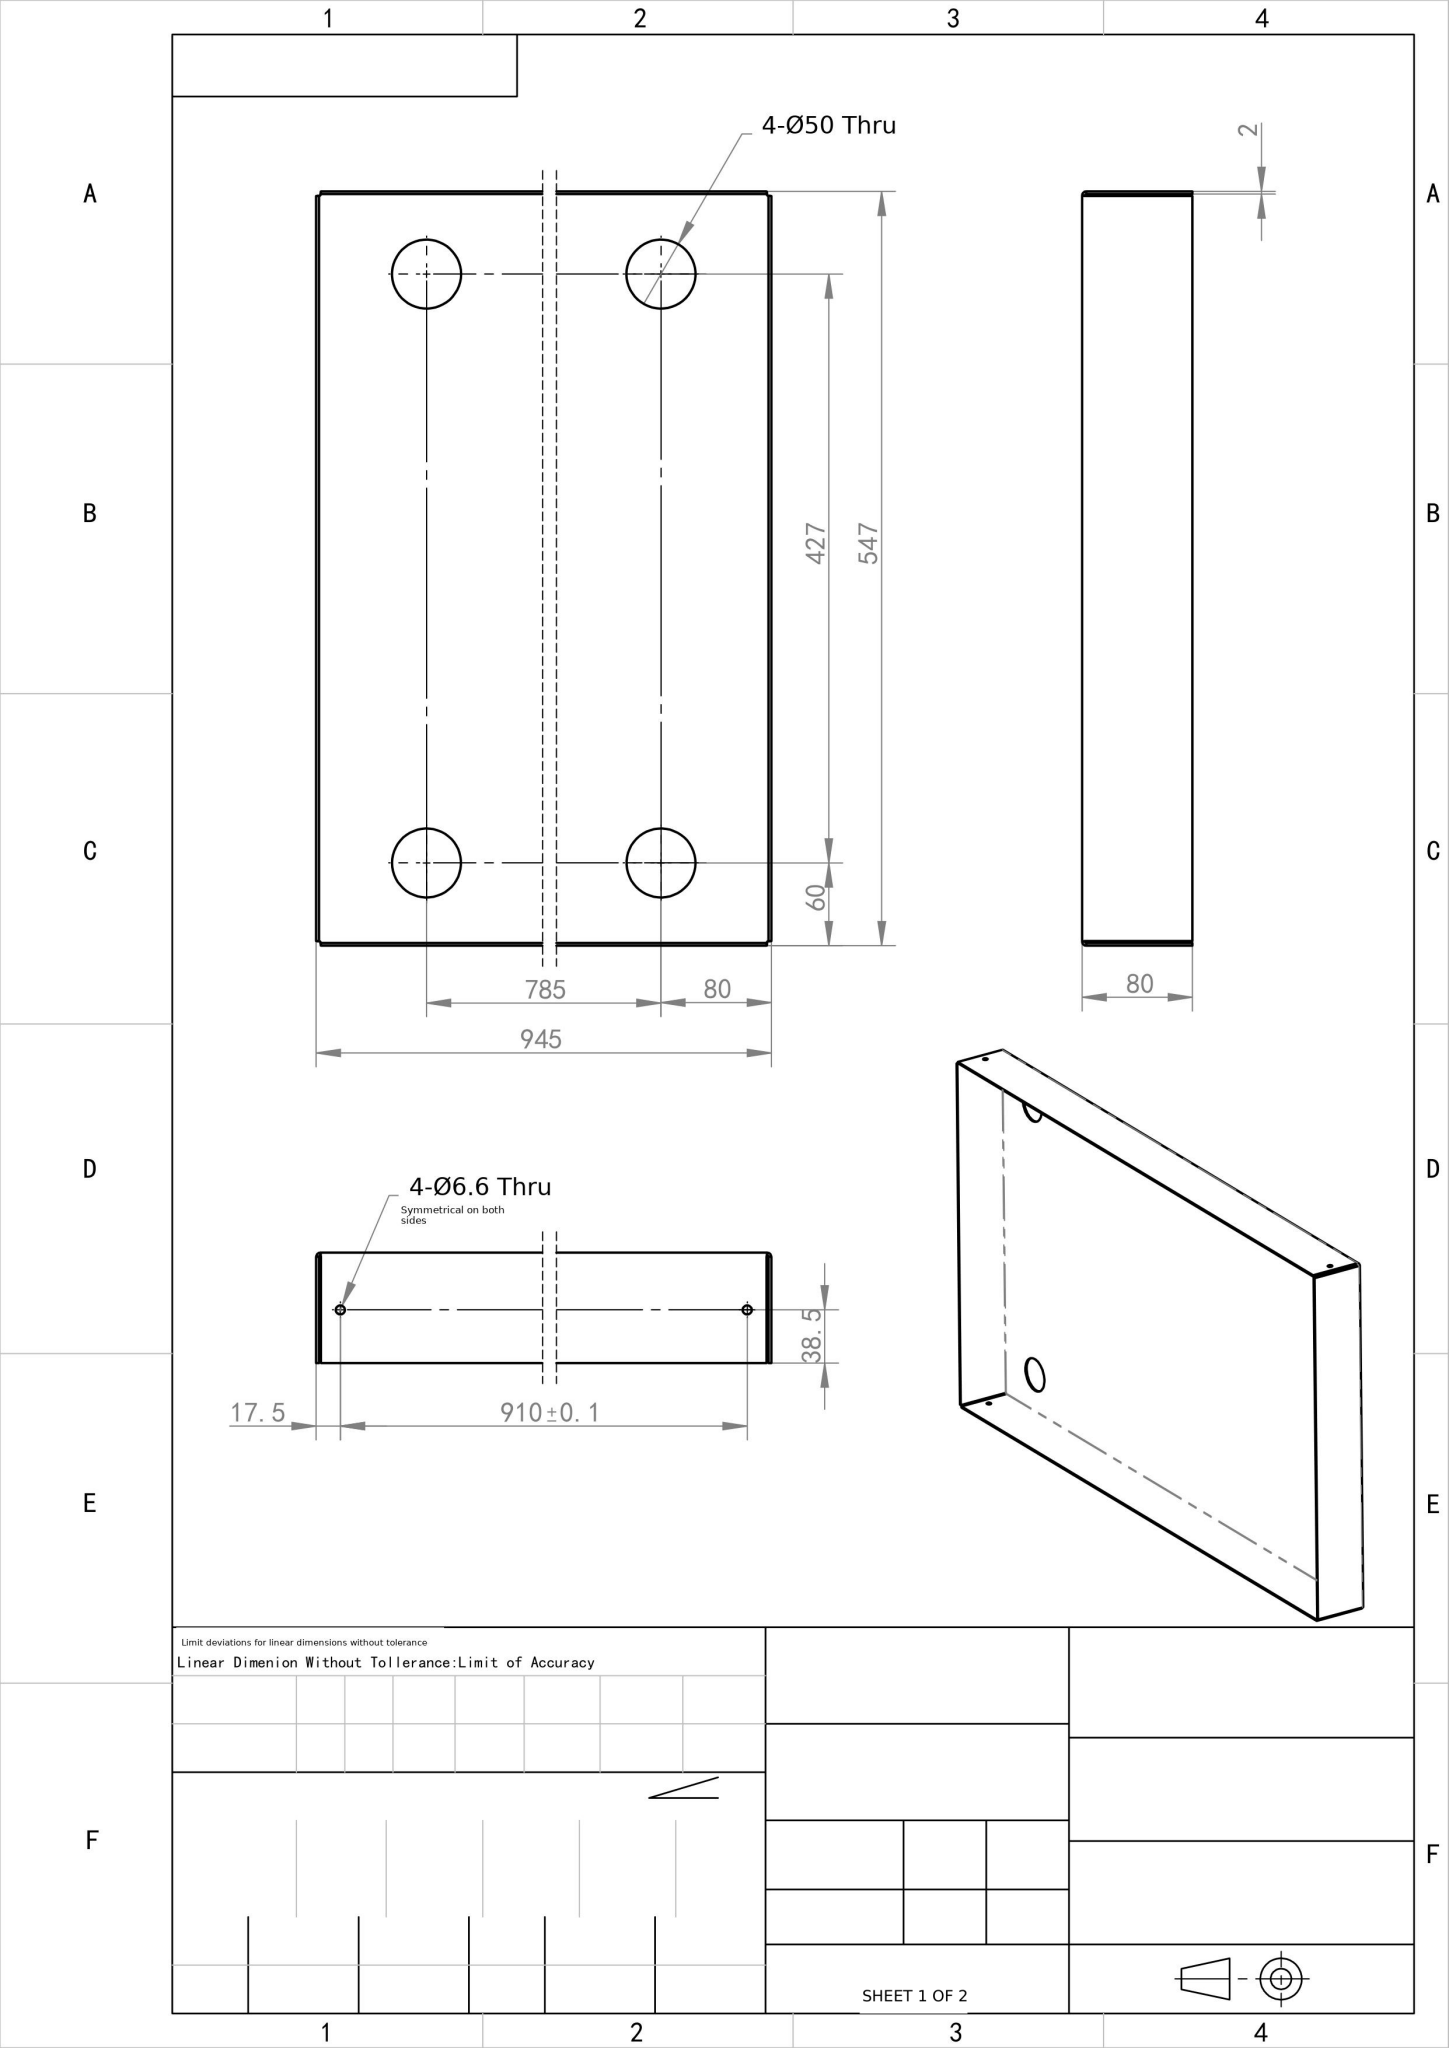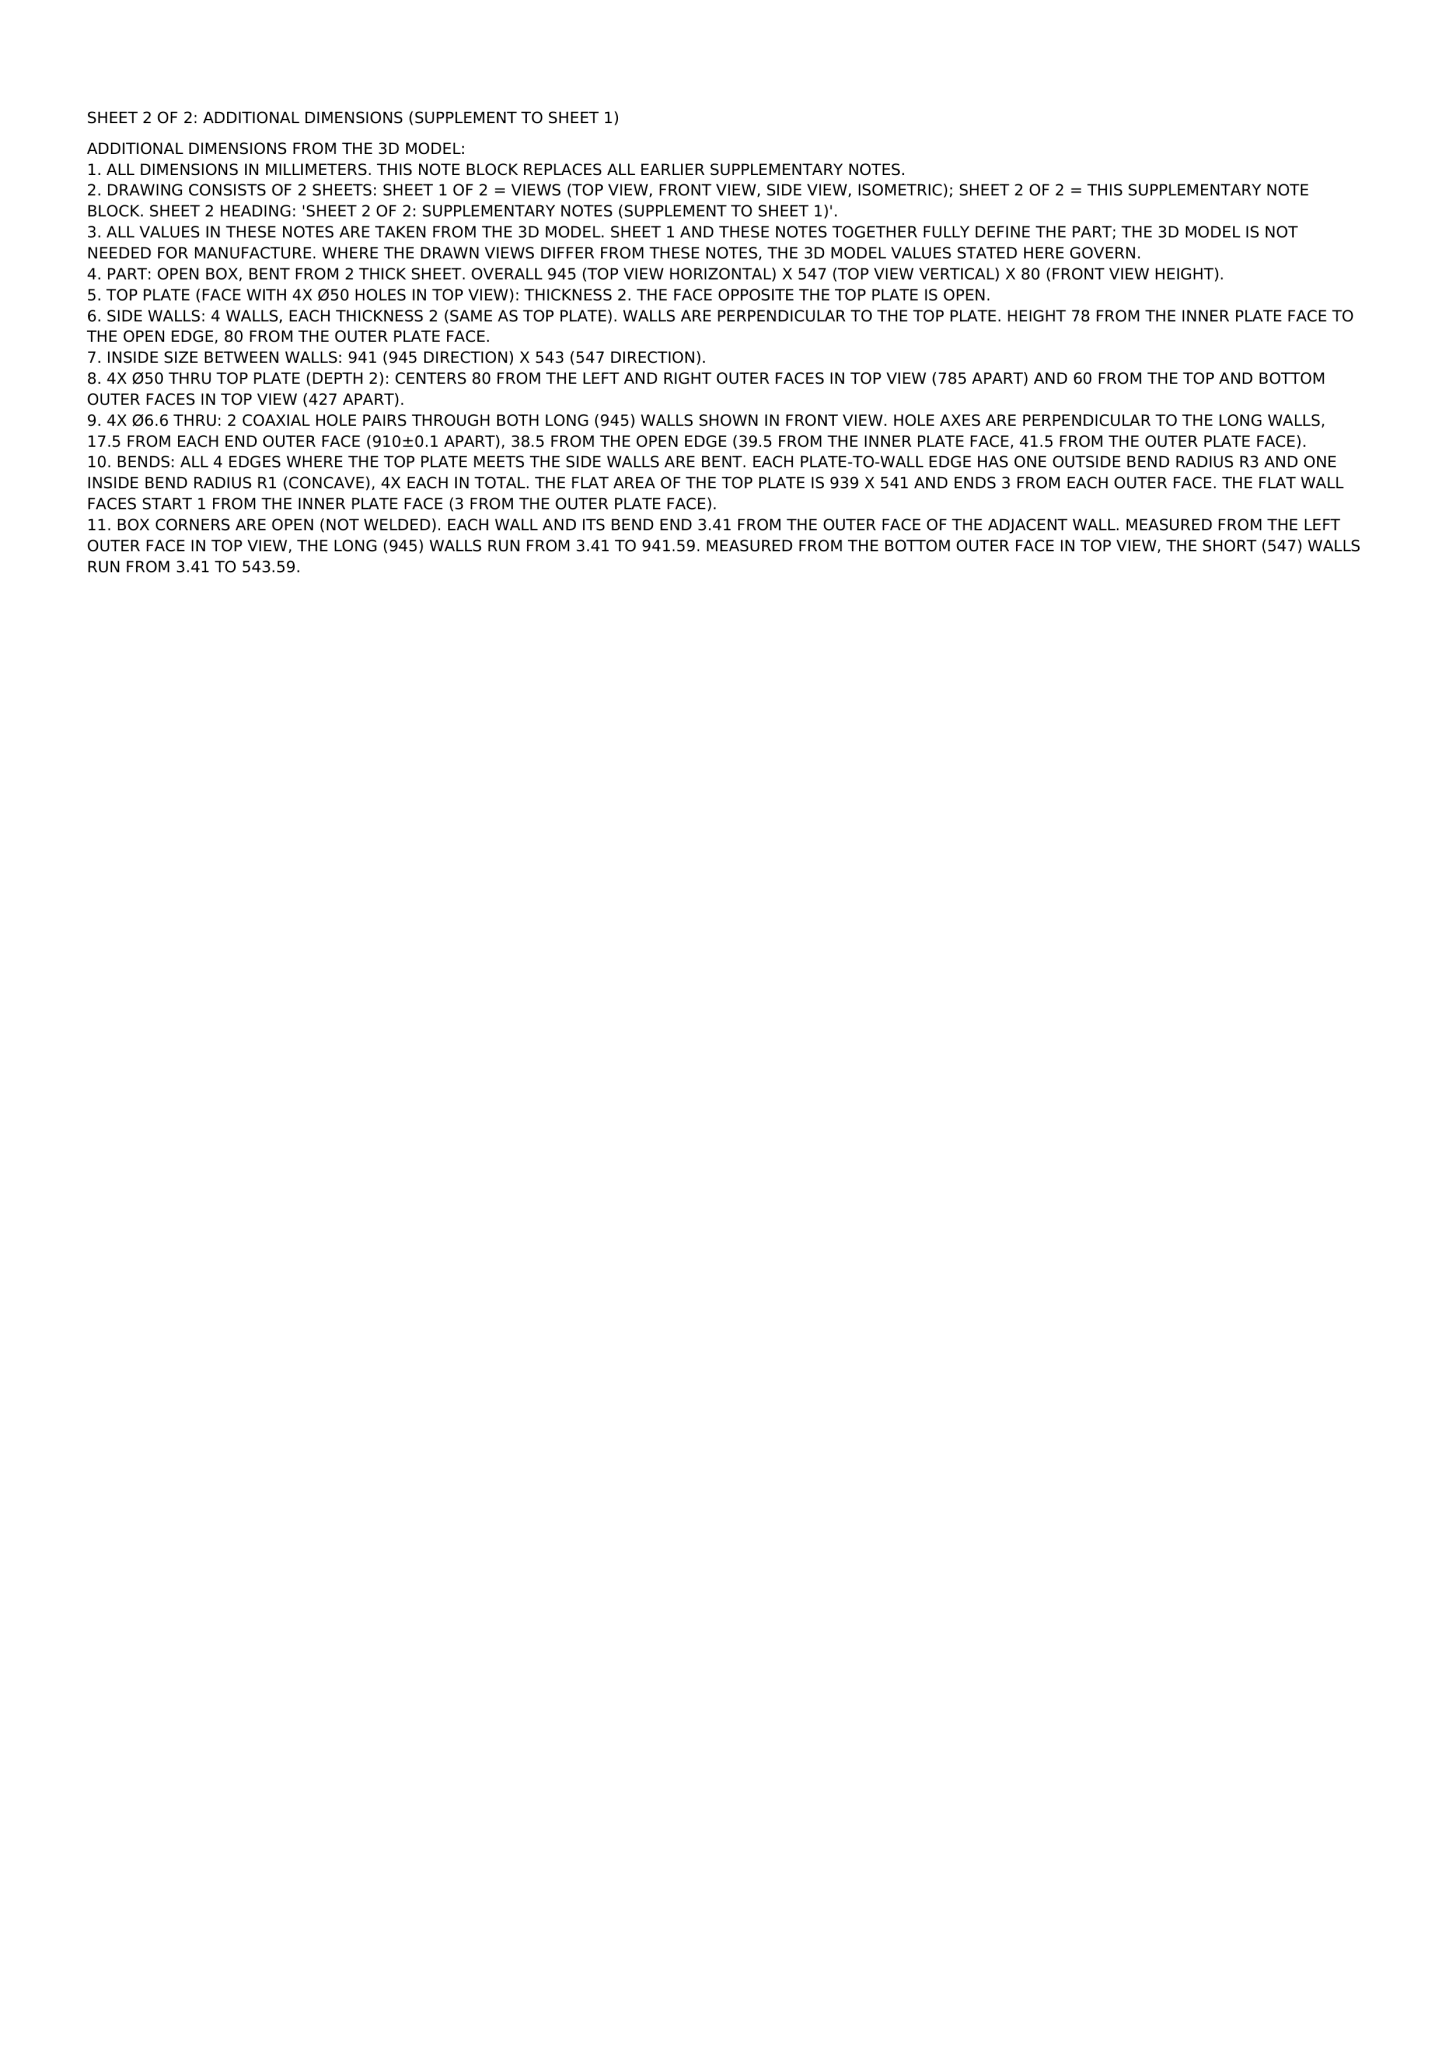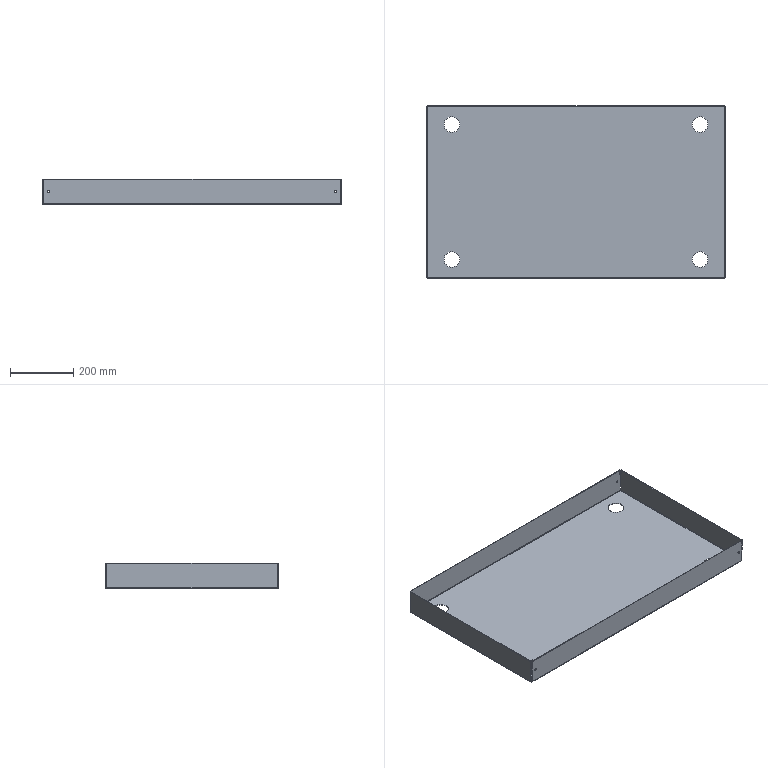Part | NX | mm | 1 solid | 54 faces | box 945 x 547 x 80 mm | volume 1473934 mm3 | cylinder 24 | plane 22 | spline 8 | commonest cylinder face diameters 6.6 x8 50 x8 6 x4 2 x4